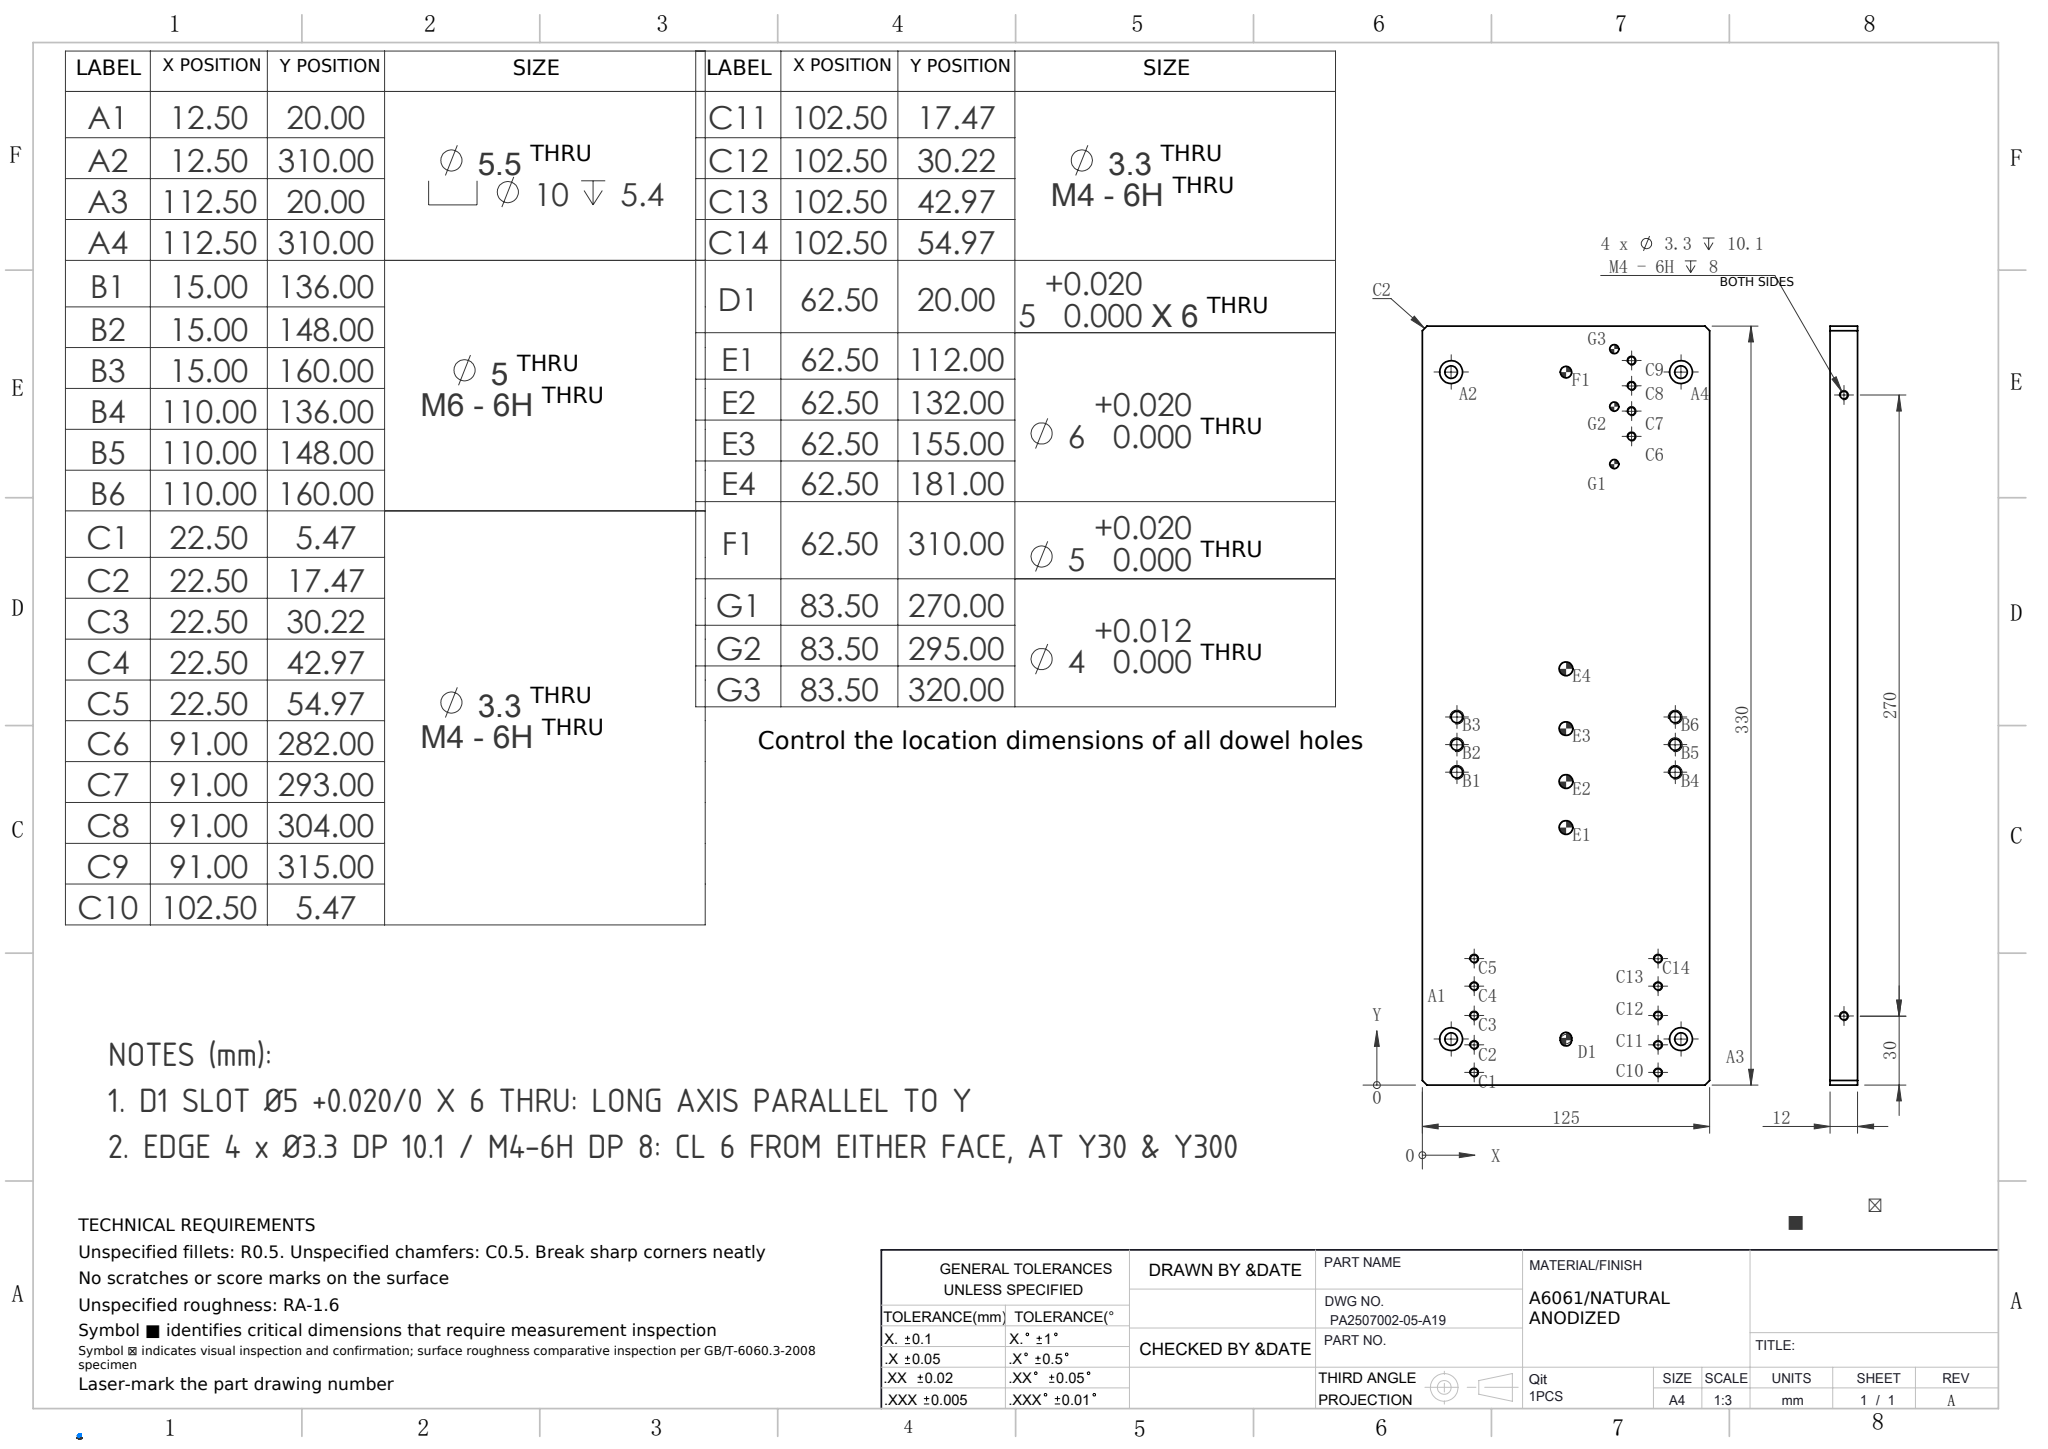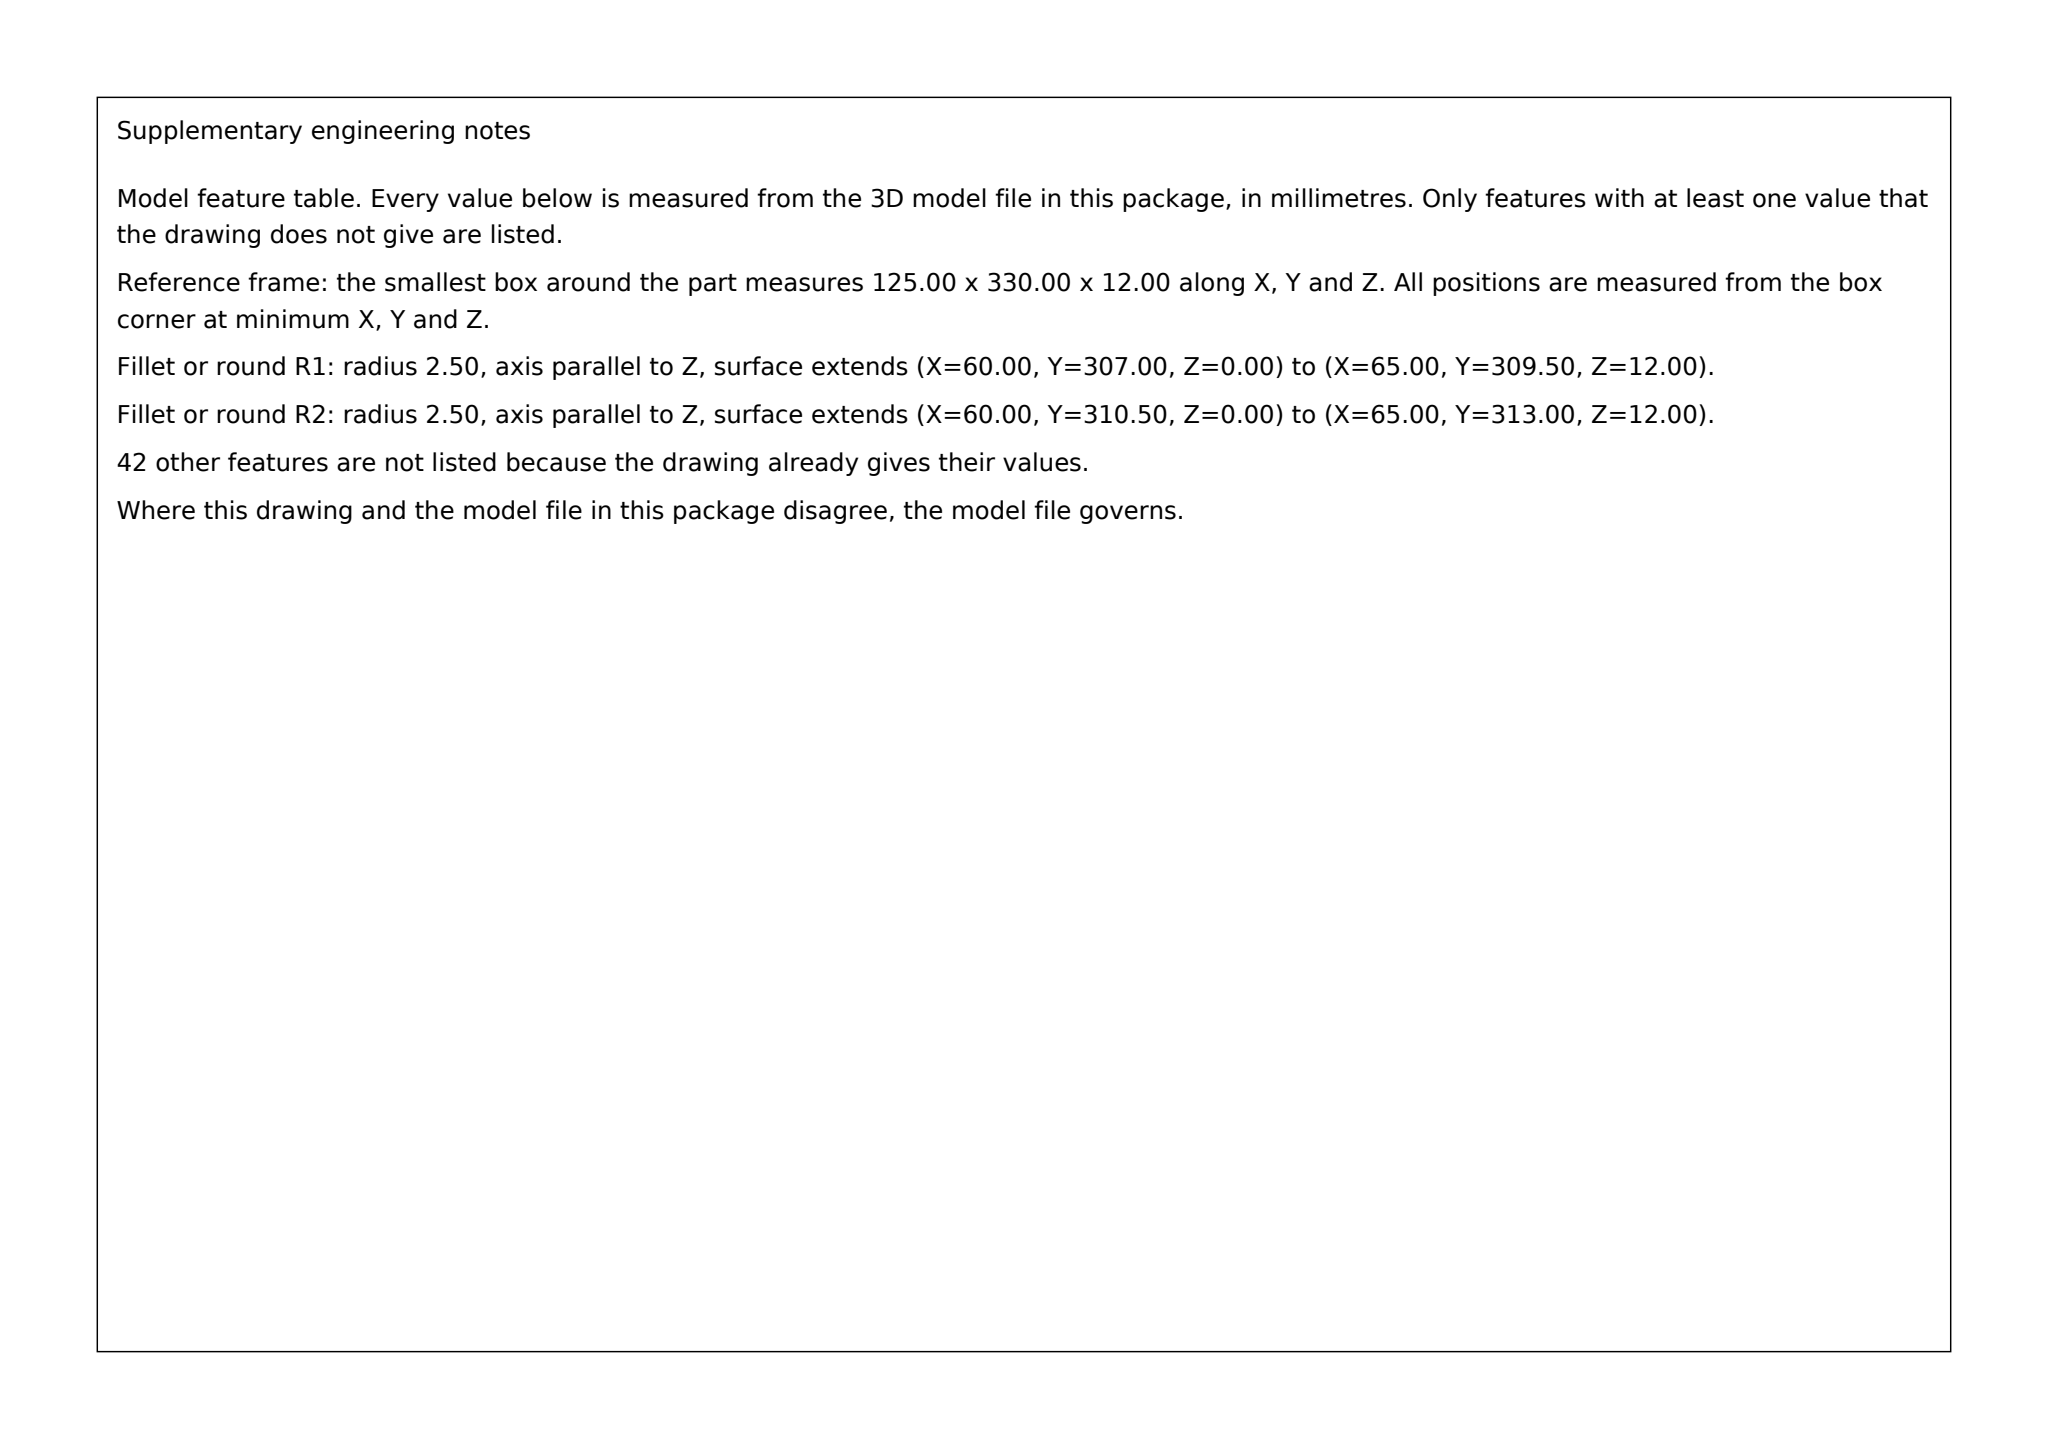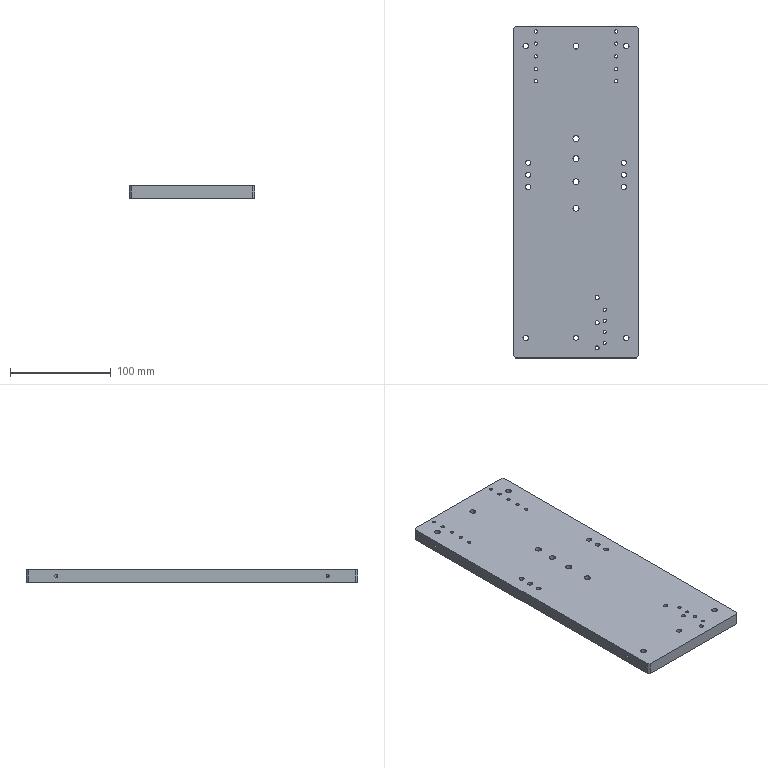Part | SolidWorks | mm | 1 solid | 106 faces | box 125 x 330 x 12 mm | volume 487032 mm3 | cylinder 82 | plane 16 | cone 8 | commonest cylinder face diameters 3.3 x36 5 x16 10 x8 5.5 x8 6 x8 4 x6
Drawing notes:
D1 SLOT Ø5 +0.020/0 X 6 THRU: LONG AXIS PARALLEL TO Y | from the solid: Ø5 end radii at (62.5,309.5) & (62.5,310.5), 1.0 apart along Y => 6 overall along Y
EDGE 4 x Ø3.3 DP 10.1 / M4-6H DP 8: CL 6 FROM EITHER FACE, AT Y30 & Y300 | from the solid: Ø3.3 x-axis holes at z=6.0 in 12.0 thick plate (bbox z=12), y=30 & y=300